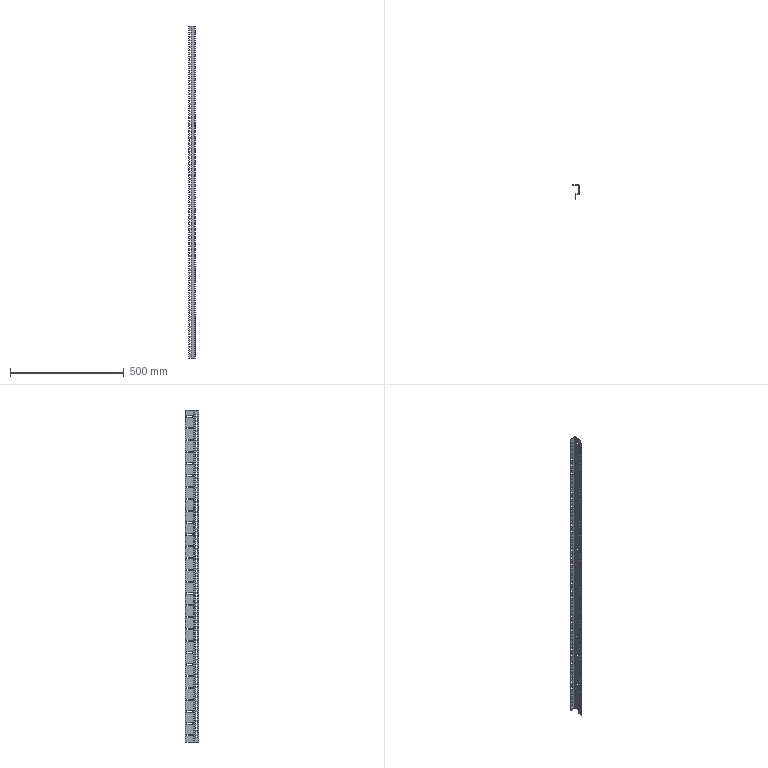Component | SolidWorks | SmallColumn-1 | 1 solid | 1066 faces | volume 254727 mm3 | plane 912 | cylinder 154 | commonest cylinder face diameters 6 x87 2 x35 1 x32